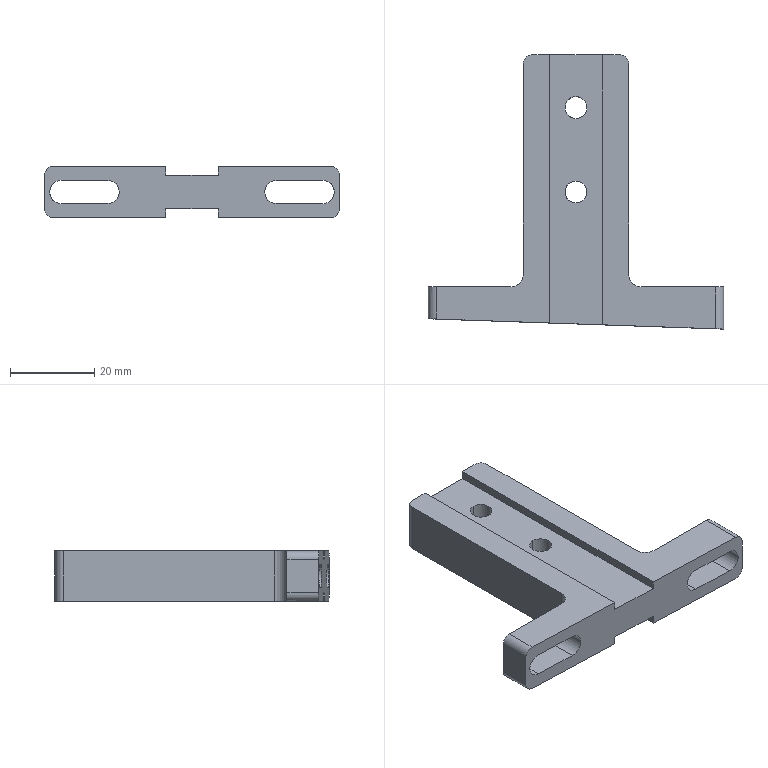CAM job | Mastercam | mm | 15 operations | part box 70 x 65 x 12
1. Facing | 20 - 63 平铣刀
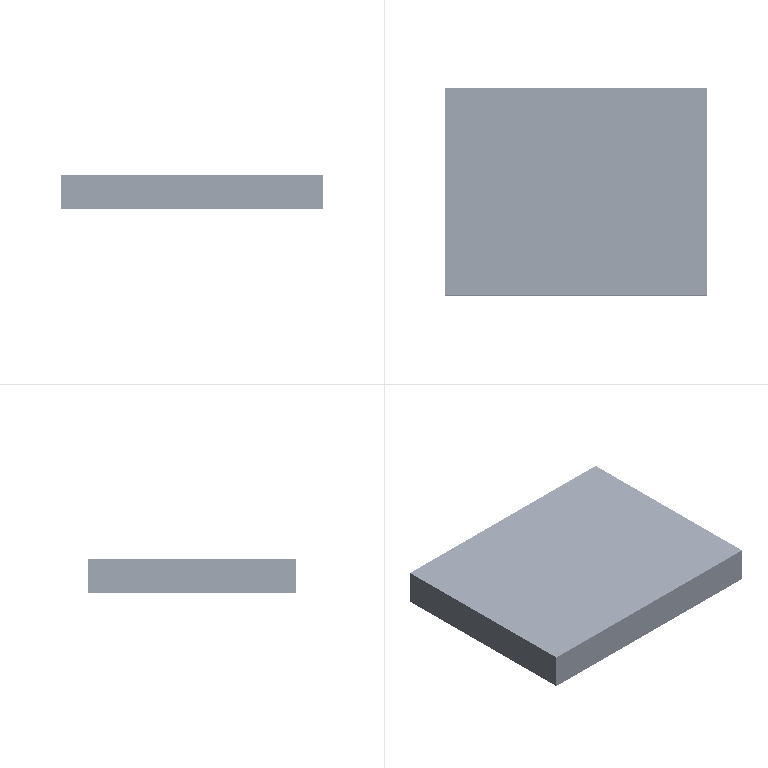2. 2D High Speed (2D Dynamic Mill) | 10 - 10 平铣刀
3. Contour (Ramp) | 10 - 10 平铣刀
4. Contour (2D) | 10 - 10 平铣刀
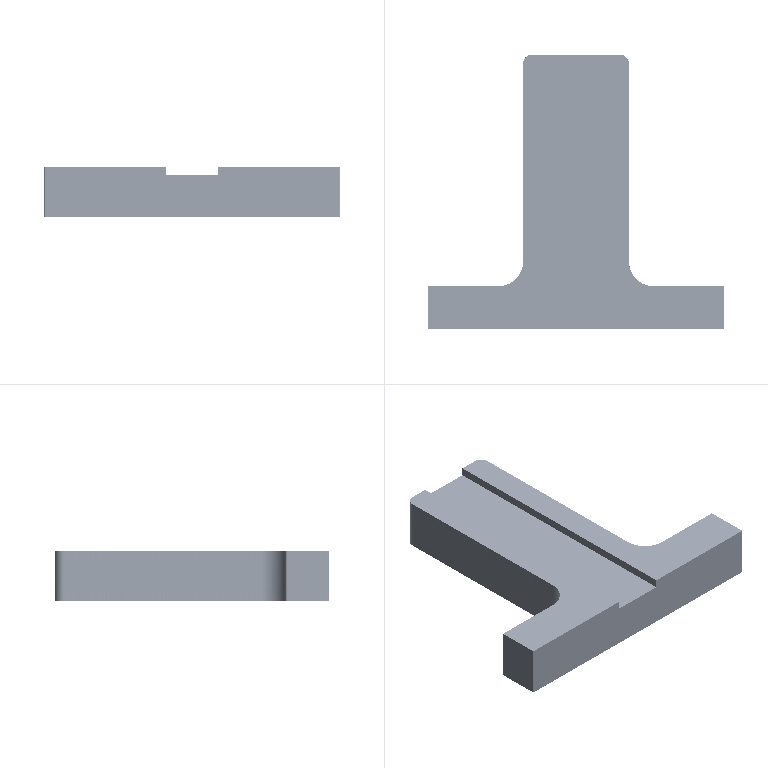5. Contour (Remachining) | 6 - 6 平铣刀
6. Contour (2D) | 6 - 6 平铣刀
7. Drill/Counterbore | 7 - 4 倒角刀
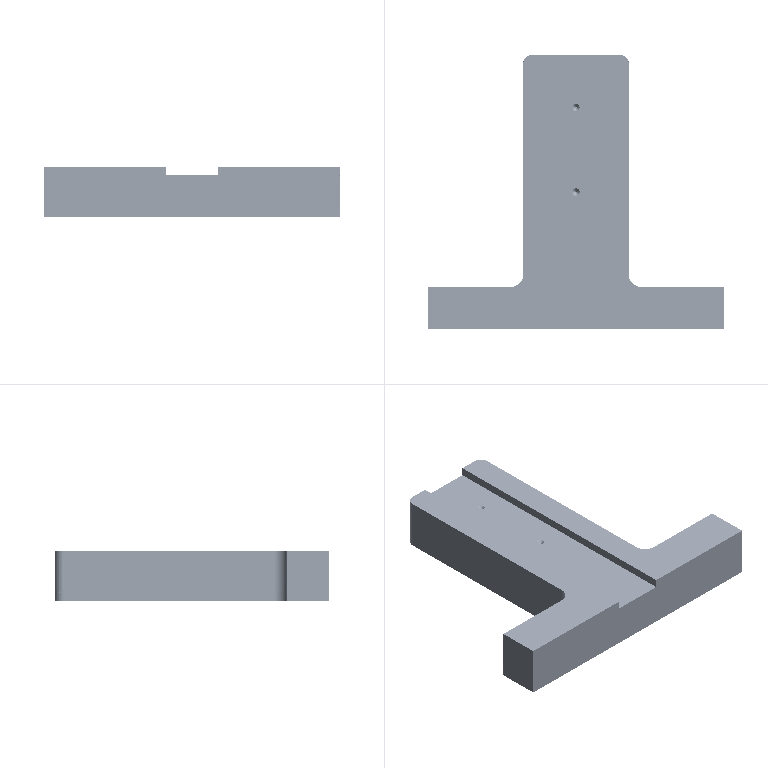8. Contour (2D chamfer) | 7 - 4 倒角刀
9. Contour (2D chamfer) | 7 - 4 倒角刀
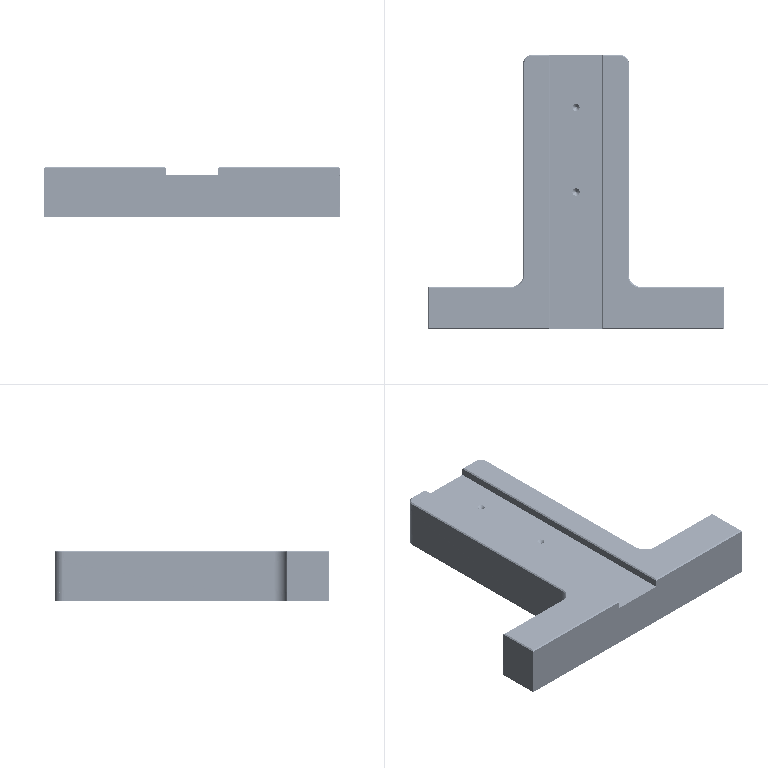10. Contour (2D) | 10 - 10 平铣刀
11. Facing | 20 - 63 平铣刀
12. Contour (Ramp) | 10 - 10 平铣刀
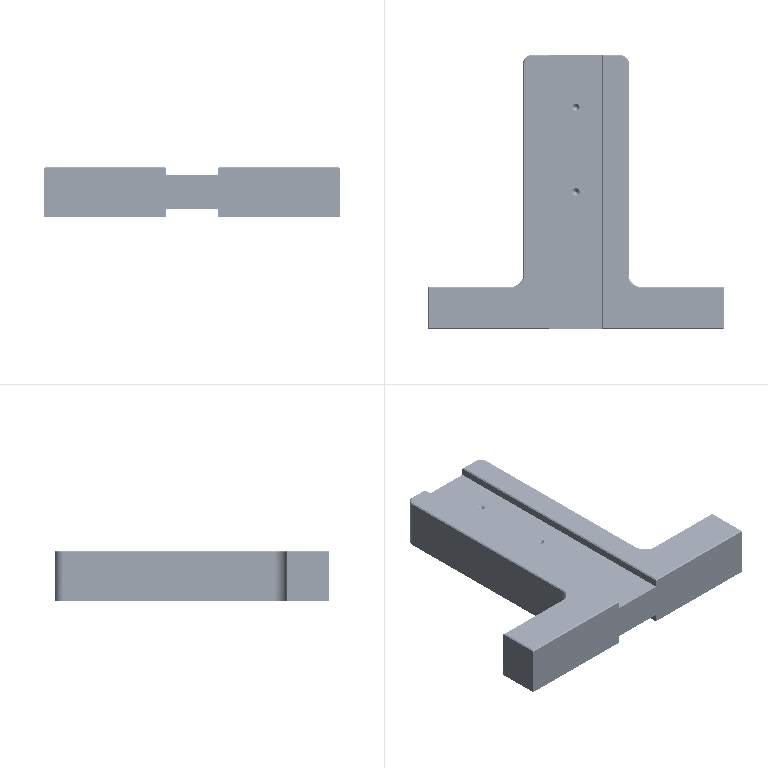13. Contour (2D) | 10 - 10 平铣刀
14. Contour (2D chamfer) | 7 - 4 倒角刀
15. Contour (2D chamfer) | 7 - 4 倒角刀